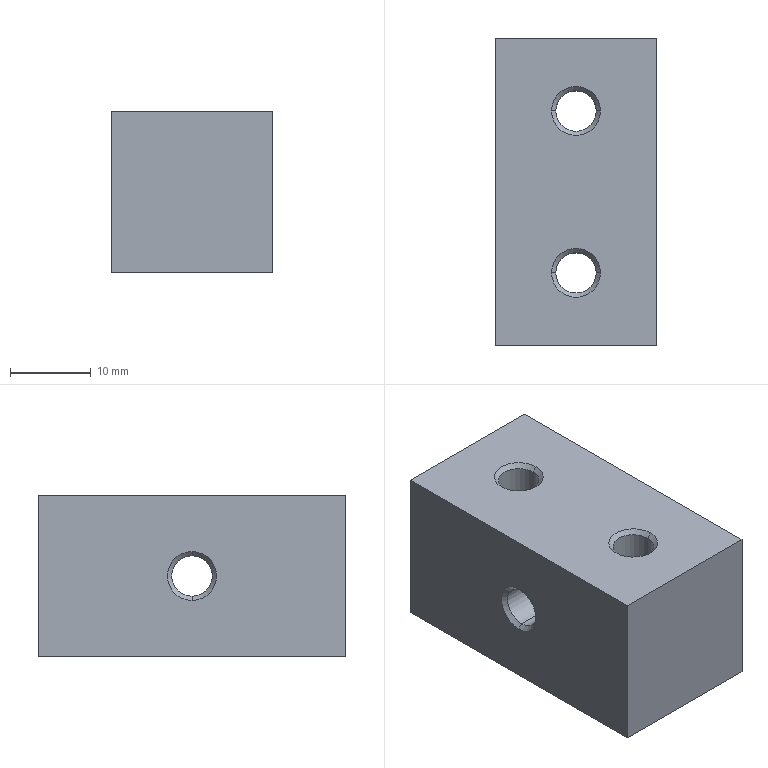Component | SolidWorks | NameDuplicate-1SupportBlock-2 | 1 solid | 18 faces | box 20 x 38 x 20 mm | volume 14015 mm3 | cone 6 | cylinder 6 | plane 6 | commonest cylinder face diameters 5 x6
build123d program:
from build123d import *

# Parameters (mm, degrees)
SKETCH1_W                = 20
SKETCH1_H                = 38
BOSS_EXTRUDE1_DEPTH      = 20
F_5_0_5_DIAMETER_HOLE1_D = 5
F_5_0_5_DIAMETER_HOLE2_D = 5
CHAMFER1_SIZE            = 0.525


with BuildPart() as part:
    # Sketch1 → Boss-Extrude1 (new body)
    with BuildSketch(Plane(origin=(10, 0, 0), x_dir=(0, 0, -1), z_dir=(1, 0, 0))):
        Rectangle(SKETCH1_W, SKETCH1_H)
    extrude(amount=-BOSS_EXTRUDE1_DEPTH)

    # 5.0 _5_ Diameter Hole1 (through all)
    with Locations(Plane(origin=(10, 0, 0), x_dir=(0, 0, -1), z_dir=(1, 0, 0))):
        with Locations((0, 0)):
            Hole(F_5_0_5_DIAMETER_HOLE1_D / 2)

    # 5.0 _5_ Diameter Hole2 (through all)
    with Locations(Plane.XY.offset(10)):
        with Locations((0, -10), (0, 10)):
            Hole(F_5_0_5_DIAMETER_HOLE2_D / 2)

    # Chamfer1
    chamfer1_edges = [part.edges().sort_by_distance(p)[0] for p in [
        (10, 0, -2.5),
        (2.5, 10, 10),
        (2.5, -10, 10),
    ]]
    chamfer(chamfer1_edges, length=CHAMFER1_SIZE)


solid = part.part

# Placed as in the assembly
solid = solid.moved(Location((-387, 406, -252.5), (0, 0, 180)))
STEP:
#1=COLOUR_RGB('',0.7922,0.8196,0.9333);
#2=FILL_AREA_STYLE_COLOUR('',#1);
#3=FILL_AREA_STYLE('',(#2));
#4=SURFACE_STYLE_FILL_AREA(#3);
#5=SURFACE_SIDE_STYLE('',(#4));
#6=SURFACE_STYLE_USAGE(.BOTH.,#5);
#7=PRESENTATION_STYLE_ASSIGNMENT((#6));
#8=CARTESIAN_POINT('',(-15.138,16.378,-9.568));
#9=VERTEX_POINT('',#8);
#10=CARTESIAN_POINT('',(-15.335,16.378,-9.568));
#11=VERTEX_POINT('',#10);
#12=CARTESIAN_POINT('',(-15.236,16.378,-9.568));
#13=DIRECTION('',(0.,0.,1.));
#14=DIRECTION('',(-1.,0.,0.));
#15=AXIS2_PLACEMENT_3D('',#12,#13,#14);
#16=CIRCLE('',#15,0.09843);
#17=EDGE_CURVE('',#9,#11,#16,.T.);
#18=ORIENTED_EDGE('',*,*,#17,.F.);
#19=CARTESIAN_POINT('',(-15.117,16.378,-9.547));
#20=VERTEX_POINT('',#19);
#21=CARTESIAN_POINT('',(-15.138,16.378,-9.568));
#22=DIRECTION('',(0.7071,0.,0.7071));
#23=VECTOR('',#22,39.37);
#24=LINE('',#21,#23);
#25=EDGE_CURVE('',#9,#20,#24,.T.);
#26=ORIENTED_EDGE('',*,*,#25,.T.);
#27=CARTESIAN_POINT('',(-15.355,16.378,-9.547));
#28=VERTEX_POINT('',#27);
#29=CARTESIAN_POINT('',(-15.236,16.378,-9.547));
#30=DIRECTION('',(-0.,-0.,-1.));
#31=DIRECTION('',(-1.,0.,0.));
#32=AXIS2_PLACEMENT_3D('',#29,#30,#31);
#33=CIRCLE('',#32,0.1191);
#34=EDGE_CURVE('',#28,#20,#33,.T.);
#35=ORIENTED_EDGE('',*,*,#34,.F.);
#36=CARTESIAN_POINT('',(-15.335,16.378,-9.568));
#37=DIRECTION('',(-0.7071,-0.,0.7071));
#38=VECTOR('',#37,39.37);
#39=LINE('',#36,#38);
#40=EDGE_CURVE('',#11,#28,#39,.T.);
#41=ORIENTED_EDGE('',*,*,#40,.F.);
#42=EDGE_LOOP('',(#18,#26,#35,#41));
#43=FACE_OUTER_BOUND('',#42,.T.);
#44=CARTESIAN_POINT('',(-15.236,16.378,-9.568));
#45=DIRECTION('',(0.,0.,1.));
#46=DIRECTION('',(-1.,0.,0.));
#47=AXIS2_PLACEMENT_3D('',#44,#45,#46);
#48=CONICAL_SURFACE('',#47,0.09843,0.7854);
#49=ADVANCED_FACE('',(#43),#48,.F.);
#50=CARTESIAN_POINT('',(-15.609,15.984,-9.843));
#51=VERTEX_POINT('',#50);
#52=CARTESIAN_POINT('',(-15.609,15.984,-10.039));
#53=VERTEX_POINT('',#52);
#54=CARTESIAN_POINT('',(-15.609,15.984,-9.941));
#55=DIRECTION('',(-1.,-0.,0.));
#56=DIRECTION('',(0.,0.,-1.));
#57=AXIS2_PLACEMENT_3D('',#54,#55,#56);
#58=CIRCLE('',#57,0.09843);
#59=EDGE_CURVE('',#51,#53,#58,.T.);
#60=ORIENTED_EDGE('',*,*,#59,.F.);
#61=CARTESIAN_POINT('',(-15.63,15.984,-9.822));
#62=VERTEX_POINT('',#61);
#63=CARTESIAN_POINT('',(-15.609,15.984,-9.843));
#64=DIRECTION('',(-0.7071,-0.,0.7071));
#65=VECTOR('',#64,39.37);
#66=LINE('',#63,#65);
#67=EDGE_CURVE('',#51,#62,#66,.T.);
#68=ORIENTED_EDGE('',*,*,#67,.T.);
#69=CARTESIAN_POINT('',(-15.63,15.984,-10.06));
#70=VERTEX_POINT('',#69);
#71=CARTESIAN_POINT('',(-15.63,15.984,-9.941));
#72=DIRECTION('',(1.,0.,-0.));
#73=DIRECTION('',(0.,0.,-1.));
#74=AXIS2_PLACEMENT_3D('',#71,#72,#73);
#75=CIRCLE('',#74,0.1191);
#76=EDGE_CURVE('',#70,#62,#75,.T.);
#77=ORIENTED_EDGE('',*,*,#76,.F.);
#78=CARTESIAN_POINT('',(-15.609,15.984,-10.039));
#79=DIRECTION('',(-0.7071,-0.,-0.7071));
#80=VECTOR('',#79,39.37);
#81=LINE('',#78,#80);
#82=EDGE_CURVE('',#53,#70,#81,.T.);
#83=ORIENTED_EDGE('',*,*,#82,.F.);
#84=EDGE_LOOP('',(#60,#68,#77,#83));
#85=FACE_OUTER_BOUND('',#84,.T.);
#86=CARTESIAN_POINT('',(-15.609,15.984,-9.941));
#87=DIRECTION('',(-1.,-0.,0.));
#88=DIRECTION('',(0.,0.,-1.));
#89=AXIS2_PLACEMENT_3D('',#86,#87,#88);
#90=CONICAL_SURFACE('',#89,0.09843,0.7854);
#91=ADVANCED_FACE('',(#85),#90,.F.);
#92=CARTESIAN_POINT('',(-15.138,15.591,-9.568));
#93=VERTEX_POINT('',#92);
#94=CARTESIAN_POINT('',(-15.335,15.591,-9.568));
#95=VERTEX_POINT('',#94);
#96=CARTESIAN_POINT('',(-15.236,15.591,-9.568));
#97=DIRECTION('',(0.,0.,1.));
#98=DIRECTION('',(-1.,0.,0.));
#99=AXIS2_PLACEMENT_3D('',#96,#97,#98);
#100=CIRCLE('',#99,0.09843);
#101=EDGE_CURVE('',#93,#95,#100,.T.);
#102=ORIENTED_EDGE('',*,*,#101,.F.);
#103=CARTESIAN_POINT('',(-15.117,15.591,-9.547));
#104=VERTEX_POINT('',#103);
#105=CARTESIAN_POINT('',(-15.138,15.591,-9.568));
#106=DIRECTION('',(0.7071,0.,0.7071));
#107=VECTOR('',#106,39.37);
#108=LINE('',#105,#107);
#109=EDGE_CURVE('',#93,#104,#108,.T.);
#110=ORIENTED_EDGE('',*,*,#109,.T.);
#111=CARTESIAN_POINT('',(-15.355,15.591,-9.547));
#112=VERTEX_POINT('',#111);
#113=CARTESIAN_POINT('',(-15.236,15.591,-9.547));
#114=DIRECTION('',(-0.,-0.,-1.));
#115=DIRECTION('',(-1.,0.,0.));
#116=AXIS2_PLACEMENT_3D('',#113,#114,#115);
#117=CIRCLE('',#116,0.1191);
#118=EDGE_CURVE('',#112,#104,#117,.T.);
#119=ORIENTED_EDGE('',*,*,#118,.F.);
#120=CARTESIAN_POINT('',(-15.335,15.591,-9.568));
#121=DIRECTION('',(-0.7071,-0.,0.7071));
#122=VECTOR('',#121,39.37);
#123=LINE('',#120,#122);
#124=EDGE_CURVE('',#95,#112,#123,.T.);
#125=ORIENTED_EDGE('',*,*,#124,.F.);
#126=EDGE_LOOP('',(#102,#110,#119,#125));
#127=FACE_OUTER_BOUND('',#126,.T.);
#128=CARTESIAN_POINT('',(-15.236,15.591,-9.568));
#129=DIRECTION('',(0.,0.,1.));
#130=DIRECTION('',(-1.,0.,0.));
#131=AXIS2_PLACEMENT_3D('',#128,#129,#130);
#132=CONICAL_SURFACE('',#131,0.09843,0.7854);
#133=ADVANCED_FACE('',(#127),#132,.F.);
#134=CARTESIAN_POINT('',(-15.138,16.378,-10.335));
#135=VERTEX_POINT('',#134);
#136=CARTESIAN_POINT('',(-15.335,16.378,-10.335));
#137=VERTEX_POINT('',#136);
#138=CARTESIAN_POINT('',(-15.236,16.378,-10.335));
#139=DIRECTION('',(0.,0.,1.));
#140=DIRECTION('',(-1.,0.,0.));
#141=AXIS2_PLACEMENT_3D('',#138,#139,#140);
#142=CIRCLE('',#141,0.09843);
#143=EDGE_CURVE('',#135,#137,#142,.T.);
#144=ORIENTED_EDGE('',*,*,#143,.F.);
#145=CARTESIAN_POINT('',(-15.138,16.378,-9.547));
#146=DIRECTION('',(0.,0.,1.));
#147=VECTOR('',#146,39.37);
#148=LINE('',#145,#147);
#149=EDGE_CURVE('',#135,#9,#148,.T.);
#150=ORIENTED_EDGE('',*,*,#149,.T.);
#151=ORIENTED_EDGE('',*,*,#17,.T.);
#152=CARTESIAN_POINT('',(-15.335,16.378,-9.547));
#153=DIRECTION('',(0.,0.,1.));
#154=VECTOR('',#153,39.37);
#155=LINE('',#152,#154);
#156=EDGE_CURVE('',#137,#11,#155,.T.);
#157=ORIENTED_EDGE('',*,*,#156,.F.);
#158=EDGE_LOOP('',(#144,#150,#151,#157));
#159=FACE_OUTER_BOUND('',#158,.T.);
#160=CARTESIAN_POINT('',(-15.236,16.378,-9.547));
#161=DIRECTION('',(0.,0.,1.));
#162=DIRECTION('',(-1.,0.,0.));
#163=AXIS2_PLACEMENT_3D('',#160,#161,#162);
#164=CYLINDRICAL_SURFACE('',#163,0.09843);
#165=ADVANCED_FACE('',(#159),#164,.F.);
#166=CARTESIAN_POINT('',(-15.138,15.591,-10.335));
#167=VERTEX_POINT('',#166);
#168=CARTESIAN_POINT('',(-15.335,15.591,-10.335));
#169=VERTEX_POINT('',#168);
#170=CARTESIAN_POINT('',(-15.236,15.591,-10.335));
#171=DIRECTION('',(0.,0.,1.));
#172=DIRECTION('',(-1.,0.,0.));
#173=AXIS2_PLACEMENT_3D('',#170,#171,#172);
#174=CIRCLE('',#173,0.09843);
#175=EDGE_CURVE('',#167,#169,#174,.T.);
#176=ORIENTED_EDGE('',*,*,#175,.F.);
#177=CARTESIAN_POINT('',(-15.138,15.591,-9.547));
#178=DIRECTION('',(0.,0.,1.));
#179=VECTOR('',#178,39.37);
#180=LINE('',#177,#179);
#181=EDGE_CURVE('',#167,#93,#180,.T.);
#182=ORIENTED_EDGE('',*,*,#181,.T.);
#183=ORIENTED_EDGE('',*,*,#101,.T.);
#184=CARTESIAN_POINT('',(-15.335,15.591,-9.547));
#185=DIRECTION('',(0.,0.,1.));
#186=VECTOR('',#185,39.37);
#187=LINE('',#184,#186);
#188=EDGE_CURVE('',#169,#95,#187,.T.);
#189=ORIENTED_EDGE('',*,*,#188,.F.);
#190=EDGE_LOOP('',(#176,#182,#183,#189));
#191=FACE_OUTER_BOUND('',#190,.T.);
#192=CARTESIAN_POINT('',(-15.236,15.591,-9.547));
#193=DIRECTION('',(0.,0.,1.));
#194=DIRECTION('',(-1.,0.,0.));
#195=AXIS2_PLACEMENT_3D('',#192,#193,#194);
#196=CYLINDRICAL_SURFACE('',#195,0.09843);
#197=ADVANCED_FACE('',(#191),#196,.F.);
#198=CARTESIAN_POINT('',(-14.843,15.984,-9.843));
#199=VERTEX_POINT('',#198);
#200=CARTESIAN_POINT('',(-14.843,15.984,-10.039));
#201=VERTEX_POINT('',#200);
#202=CARTESIAN_POINT('',(-14.843,15.984,-9.941));
#203=DIRECTION('',(-1.,-0.,0.));
#204=DIRECTION('',(0.,0.,-1.));
#205=AXIS2_PLACEMENT_3D('',#202,#203,#204);
#206=CIRCLE('',#205,0.09843);
#207=EDGE_CURVE('',#199,#201,#206,.T.);
#208=ORIENTED_EDGE('',*,*,#207,.F.);
#209=CARTESIAN_POINT('',(-15.63,15.984,-9.843));
#210=DIRECTION('',(-1.,-0.,0.));
#211=VECTOR('',#210,39.37);
#212=LINE('',#209,#211);
#213=EDGE_CURVE('',#199,#51,#212,.T.);
#214=ORIENTED_EDGE('',*,*,#213,.T.);
#215=ORIENTED_EDGE('',*,*,#59,.T.);
#216=CARTESIAN_POINT('',(-15.63,15.984,-10.039));
#217=DIRECTION('',(-1.,-0.,0.));
#218=VECTOR('',#217,39.37);
#219=LINE('',#216,#218);
#220=EDGE_CURVE('',#201,#53,#219,.T.);
#221=ORIENTED_EDGE('',*,*,#220,.F.);
#222=EDGE_LOOP('',(#208,#214,#215,#221));
#223=FACE_OUTER_BOUND('',#222,.T.);
#224=CARTESIAN_POINT('',(-15.63,15.984,-9.941));
#225=DIRECTION('',(-1.,-0.,0.));
#226=DIRECTION('',(0.,0.,-1.));
#227=AXIS2_PLACEMENT_3D('',#224,#225,#226);
#228=CYLINDRICAL_SURFACE('',#227,0.09843);
#229=ADVANCED_FACE('',(#223),#228,.F.);
#230=CARTESIAN_POINT('',(-15.63,15.236,-10.335));
#231=VERTEX_POINT('',#230);
#232=CARTESIAN_POINT('',(-15.63,15.236,-9.547));
#233=VERTEX_POINT('',#232);
#234=CARTESIAN_POINT('',(-15.63,15.236,-10.335));
#235=DIRECTION('',(0.,0.,1.));
#236=VECTOR('',#235,39.37);
#237=LINE('',#234,#236);
#238=EDGE_CURVE('',#231,#233,#237,.T.);
#239=ORIENTED_EDGE('',*,*,#238,.F.);
#240=CARTESIAN_POINT('',(-14.843,15.236,-10.335));
#241=VERTEX_POINT('',#240);
#242=CARTESIAN_POINT('',(-14.843,15.236,-10.335));
#243=DIRECTION('',(-1.,-0.,0.));
#244=VECTOR('',#243,39.37);
#245=LINE('',#242,#244);
#246=EDGE_CURVE('',#241,#231,#245,.T.);
#247=ORIENTED_EDGE('',*,*,#246,.F.);
#248=CARTESIAN_POINT('',(-14.843,15.236,-9.547));
#249=VERTEX_POINT('',#248);
#250=CARTESIAN_POINT('',(-14.843,15.236,-10.335));
#251=DIRECTION('',(0.,0.,1.));
#252=VECTOR('',#251,39.37);
#253=LINE('',#250,#252);
#254=EDGE_CURVE('',#241,#249,#253,.T.);
#255=ORIENTED_EDGE('',*,*,#254,.T.);
#256=CARTESIAN_POINT('',(-14.843,15.236,-9.547));
#257=DIRECTION('',(-1.,-0.,0.));
#258=VECTOR('',#257,39.37);
#259=LINE('',#256,#258);
#260=EDGE_CURVE('',#249,#233,#259,.T.);
#261=ORIENTED_EDGE('',*,*,#260,.T.);
#262=EDGE_LOOP('',(#239,#247,#255,#261));
#263=FACE_OUTER_BOUND('',#262,.T.);
#264=CARTESIAN_POINT('',(-14.843,15.236,-10.335));
#265=DIRECTION('',(0.,-1.,0.));
#266=DIRECTION('',(0.,0.,1.));
#267=AXIS2_PLACEMENT_3D('',#264,#265,#266);
#268=PLANE('',#267);
#269=ADVANCED_FACE('',(#263),#268,.T.);
#270=CARTESIAN_POINT('',(-15.236,16.378,-10.335));
#271=DIRECTION('',(0.,0.,1.));
#272=DIRECTION('',(-1.,0.,0.));
#273=AXIS2_PLACEMENT_3D('',#270,#271,#272);
#274=CIRCLE('',#273,0.09843);
#275=EDGE_CURVE('',#137,#135,#274,.T.);
#276=ORIENTED_EDGE('',*,*,#275,.T.);
#277=ORIENTED_EDGE('',*,*,#143,.T.);
#278=EDGE_LOOP('',(#276,#277));
#279=FACE_BOUND('',#278,.T.);
#280=CARTESIAN_POINT('',(-15.236,15.591,-10.335));
#281=DIRECTION('',(0.,0.,1.));
#282=DIRECTION('',(-1.,0.,0.));
#283=AXIS2_PLACEMENT_3D('',#280,#281,#282);
#284=CIRCLE('',#283,0.09843);
#285=EDGE_CURVE('',#169,#167,#284,.T.);
#286=ORIENTED_EDGE('',*,*,#285,.T.);
#287=ORIENTED_EDGE('',*,*,#175,.T.);
#288=EDGE_LOOP('',(#286,#287));
#289=FACE_BOUND('',#288,.T.);
#290=CARTESIAN_POINT('',(-15.63,16.732,-10.335));
#291=VERTEX_POINT('',#290);
#292=CARTESIAN_POINT('',(-15.63,16.732,-10.335));
#293=DIRECTION('',(0.,-1.,0.));
#294=VECTOR('',#293,39.37);
#295=LINE('',#292,#294);
#296=EDGE_CURVE('',#291,#231,#295,.T.);
#297=ORIENTED_EDGE('',*,*,#296,.F.);
#298=CARTESIAN_POINT('',(-14.843,16.732,-10.335));
#299=VERTEX_POINT('',#298);
#300=CARTESIAN_POINT('',(-14.843,16.732,-10.335));
#301=DIRECTION('',(-1.,-0.,0.));
#302=VECTOR('',#301,39.37);
#303=LINE('',#300,#302);
#304=EDGE_CURVE('',#299,#291,#303,.T.);
#305=ORIENTED_EDGE('',*,*,#304,.F.);
#306=CARTESIAN_POINT('',(-14.843,16.732,-10.335));
#307=DIRECTION('',(0.,-1.,0.));
#308=VECTOR('',#307,39.37);
#309=LINE('',#306,#308);
#310=EDGE_CURVE('',#299,#241,#309,.T.);
#311=ORIENTED_EDGE('',*,*,#310,.T.);
#312=ORIENTED_EDGE('',*,*,#246,.T.);
#313=EDGE_LOOP('',(#297,#305,#311,#312));
#314=FACE_OUTER_BOUND('',#313,.T.);
#315=CARTESIAN_POINT('',(-14.843,16.732,-10.335));
#316=DIRECTION('',(-0.,-0.,-1.));
#317=DIRECTION('',(1.,0.,-0.));
#318=AXIS2_PLACEMENT_3D('',#315,#316,#317);
#319=PLANE('',#318);
#320=ADVANCED_FACE('',(#279,#289,#314),#319,.T.);
#321=CARTESIAN_POINT('',(-15.63,16.732,-9.547));
#322=VERTEX_POINT('',#321);
#323=CARTESIAN_POINT('',(-15.63,16.732,-9.547));
#324=DIRECTION('',(-0.,-0.,-1.));
#325=VECTOR('',#324,39.37);
#326=LINE('',#323,#325);
#327=EDGE_CURVE('',#322,#291,#326,.T.);
#328=ORIENTED_EDGE('',*,*,#327,.F.);
#329=CARTESIAN_POINT('',(-14.843,16.732,-9.547));
#330=VERTEX_POINT('',#329);
#331=CARTESIAN_POINT('',(-14.843,16.732,-9.547));
#332=DIRECTION('',(-1.,-0.,0.));
#333=VECTOR('',#332,39.37);
#334=LINE('',#331,#333);
#335=EDGE_CURVE('',#330,#322,#334,.T.);
#336=ORIENTED_EDGE('',*,*,#335,.F.);
#337=CARTESIAN_POINT('',(-14.843,16.732,-9.547));
#338=DIRECTION('',(-0.,-0.,-1.));
#339=VECTOR('',#338,39.37);
#340=LINE('',#337,#339);
#341=EDGE_CURVE('',#330,#299,#340,.T.);
#342=ORIENTED_EDGE('',*,*,#341,.T.);
#343=ORIENTED_EDGE('',*,*,#304,.T.);
#344=EDGE_LOOP('',(#328,#336,#342,#343));
#345=FACE_OUTER_BOUND('',#344,.T.);
#346=CARTESIAN_POINT('',(-14.843,16.732,-9.547));
#347=DIRECTION('',(-0.,1.,-0.));
#348=DIRECTION('',(-0.,-0.,-1.));
#349=AXIS2_PLACEMENT_3D('',#346,#347,#348);
#350=PLANE('',#349);
#351=ADVANCED_FACE('',(#345),#350,.T.);
#352=ORIENTED_EDGE('',*,*,#118,.T.);
#353=CARTESIAN_POINT('',(-15.236,15.591,-9.547));
#354=DIRECTION('',(-0.,-0.,-1.));
#355=DIRECTION('',(-1.,0.,0.));
#356=AXIS2_PLACEMENT_3D('',#353,#354,#355);
#357=CIRCLE('',#356,0.1191);
#358=EDGE_CURVE('',#104,#112,#357,.T.);
#359=ORIENTED_EDGE('',*,*,#358,.T.);
#360=EDGE_LOOP('',(#352,#359));
#361=FACE_BOUND('',#360,.T.);
#362=ORIENTED_EDGE('',*,*,#34,.T.);
#363=CARTESIAN_POINT('',(-15.236,16.378,-9.547));
#364=DIRECTION('',(-0.,-0.,-1.));
#365=DIRECTION('',(-1.,0.,0.));
#366=AXIS2_PLACEMENT_3D('',#363,#364,#365);
#367=CIRCLE('',#366,0.1191);
#368=EDGE_CURVE('',#20,#28,#367,.T.);
#369=ORIENTED_EDGE('',*,*,#368,.T.);
#370=EDGE_LOOP('',(#362,#369));
#371=FACE_BOUND('',#370,.T.);
#372=CARTESIAN_POINT('',(-15.63,15.236,-9.547));
#373=DIRECTION('',(-0.,1.,-0.));
#374=VECTOR('',#373,39.37);
#375=LINE('',#372,#374);
#376=EDGE_CURVE('',#233,#322,#375,.T.);
#377=ORIENTED_EDGE('',*,*,#376,.F.);
#378=ORIENTED_EDGE('',*,*,#260,.F.);
#379=CARTESIAN_POINT('',(-14.843,15.236,-9.547));
#380=DIRECTION('',(-0.,1.,-0.));
#381=VECTOR('',#380,39.37);
#382=LINE('',#379,#381);
#383=EDGE_CURVE('',#249,#330,#382,.T.);
#384=ORIENTED_EDGE('',*,*,#383,.T.);
#385=ORIENTED_EDGE('',*,*,#335,.T.);
#386=EDGE_LOOP('',(#377,#378,#384,#385));
#387=FACE_OUTER_BOUND('',#386,.T.);
#388=CARTESIAN_POINT('',(-14.843,15.236,-9.547));
#389=DIRECTION('',(0.,0.,1.));
#390=DIRECTION('',(-1.,-0.,0.));
#391=AXIS2_PLACEMENT_3D('',#388,#389,#390);
#392=PLANE('',#391);
#393=ADVANCED_FACE('',(#361,#371,#387),#392,.T.);
#394=CARTESIAN_POINT('',(-14.843,15.984,-9.941));
#395=DIRECTION('',(-1.,-0.,0.));
#396=DIRECTION('',(0.,0.,-1.));
#397=AXIS2_PLACEMENT_3D('',#394,#395,#396);
#398=CIRCLE('',#397,0.09843);
#399=EDGE_CURVE('',#201,#199,#398,.T.);
#400=ORIENTED_EDGE('',*,*,#399,.T.);
#401=ORIENTED_EDGE('',*,*,#207,.T.);
#402=EDGE_LOOP('',(#400,#401));
#403=FACE_BOUND('',#402,.T.);
#404=ORIENTED_EDGE('',*,*,#254,.F.);
#405=ORIENTED_EDGE('',*,*,#310,.F.);
#406=ORIENTED_EDGE('',*,*,#341,.F.);
#407=ORIENTED_EDGE('',*,*,#383,.F.);
#408=EDGE_LOOP('',(#404,#405,#406,#407));
#409=FACE_OUTER_BOUND('',#408,.T.);
#410=CARTESIAN_POINT('',(-14.843,15.984,-9.941));
#411=DIRECTION('',(-1.,-0.,0.));
#412=DIRECTION('',(-0.,-0.,-1.));
#413=AXIS2_PLACEMENT_3D('',#410,#411,#412);
#414=PLANE('',#413);
#415=ADVANCED_FACE('',(#403,#409),#414,.F.);
#416=ORIENTED_EDGE('',*,*,#76,.T.);
#417=CARTESIAN_POINT('',(-15.63,15.984,-9.941));
#418=DIRECTION('',(1.,0.,-0.));
#419=DIRECTION('',(0.,0.,-1.));
#420=AXIS2_PLACEMENT_3D('',#417,#418,#419);
#421=CIRCLE('',#420,0.1191);
#422=EDGE_CURVE('',#62,#70,#421,.T.);
#423=ORIENTED_EDGE('',*,*,#422,.T.);
#424=EDGE_LOOP('',(#416,#423));
#425=FACE_BOUND('',#424,.T.);
#426=ORIENTED_EDGE('',*,*,#238,.T.);
#427=ORIENTED_EDGE('',*,*,#376,.T.);
#428=ORIENTED_EDGE('',*,*,#327,.T.);
#429=ORIENTED_EDGE('',*,*,#296,.T.);
#430=EDGE_LOOP('',(#426,#427,#428,#429));
#431=FACE_OUTER_BOUND('',#430,.T.);
#432=CARTESIAN_POINT('',(-15.63,15.984,-9.941));
#433=DIRECTION('',(-1.,-0.,0.));
#434=DIRECTION('',(-0.,-0.,-1.));
#435=AXIS2_PLACEMENT_3D('',#432,#433,#434);
#436=PLANE('',#435);
#437=ADVANCED_FACE('',(#425,#431),#436,.T.);
#438=ORIENTED_EDGE('',*,*,#213,.F.);
#439=ORIENTED_EDGE('',*,*,#399,.F.);
#440=ORIENTED_EDGE('',*,*,#220,.T.);
#441=CARTESIAN_POINT('',(-15.609,15.984,-9.941));
#442=DIRECTION('',(-1.,-0.,0.));
#443=DIRECTION('',(0.,0.,-1.));
#444=AXIS2_PLACEMENT_3D('',#441,#442,#443);
#445=CIRCLE('',#444,0.09843);
#446=EDGE_CURVE('',#53,#51,#445,.T.);
#447=ORIENTED_EDGE('',*,*,#446,.T.);
#448=EDGE_LOOP('',(#438,#439,#440,#447));
#449=FACE_OUTER_BOUND('',#448,.T.);
#450=CARTESIAN_POINT('',(-15.63,15.984,-9.941));
#451=DIRECTION('',(-1.,-0.,0.));
#452=DIRECTION('',(0.,0.,-1.));
#453=AXIS2_PLACEMENT_3D('',#450,#451,#452);
#454=CYLINDRICAL_SURFACE('',#453,0.09843);
#455=ADVANCED_FACE('',(#449),#454,.F.);
#456=ORIENTED_EDGE('',*,*,#181,.F.);
#457=ORIENTED_EDGE('',*,*,#285,.F.);
#458=ORIENTED_EDGE('',*,*,#188,.T.);
#459=CARTESIAN_POINT('',(-15.236,15.591,-9.568));
#460=DIRECTION('',(0.,0.,1.));
#461=DIRECTION('',(-1.,0.,0.));
#462=AXIS2_PLACEMENT_3D('',#459,#460,#461);
#463=CIRCLE('',#462,0.09843);
#464=EDGE_CURVE('',#95,#93,#463,.T.);
#465=ORIENTED_EDGE('',*,*,#464,.T.);
#466=EDGE_LOOP('',(#456,#457,#458,#465));
#467=FACE_OUTER_BOUND('',#466,.T.);
#468=CARTESIAN_POINT('',(-15.236,15.591,-9.547));
#469=DIRECTION('',(0.,0.,1.));
#470=DIRECTION('',(-1.,0.,0.));
#471=AXIS2_PLACEMENT_3D('',#468,#469,#470);
#472=CYLINDRICAL_SURFACE('',#471,0.09843);
#473=ADVANCED_FACE('',(#467),#472,.F.);
#474=ORIENTED_EDGE('',*,*,#149,.F.);
#475=ORIENTED_EDGE('',*,*,#275,.F.);
#476=ORIENTED_EDGE('',*,*,#156,.T.);
#477=CARTESIAN_POINT('',(-15.236,16.378,-9.568));
#478=DIRECTION('',(0.,0.,1.));
#479=DIRECTION('',(-1.,0.,0.));
#480=AXIS2_PLACEMENT_3D('',#477,#478,#479);
#481=CIRCLE('',#480,0.09843);
#482=EDGE_CURVE('',#11,#9,#481,.T.);
#483=ORIENTED_EDGE('',*,*,#482,.T.);
#484=EDGE_LOOP('',(#474,#475,#476,#483));
#485=FACE_OUTER_BOUND('',#484,.T.);
#486=CARTESIAN_POINT('',(-15.236,16.378,-9.547));
#487=DIRECTION('',(0.,0.,1.));
#488=DIRECTION('',(-1.,0.,0.));
#489=AXIS2_PLACEMENT_3D('',#486,#487,#488);
#490=CYLINDRICAL_SURFACE('',#489,0.09843);
#491=ADVANCED_FACE('',(#485),#490,.F.);
#492=ORIENTED_EDGE('',*,*,#109,.F.);
#493=ORIENTED_EDGE('',*,*,#464,.F.);
#494=ORIENTED_EDGE('',*,*,#124,.T.);
#495=ORIENTED_EDGE('',*,*,#358,.F.);
#496=EDGE_LOOP('',(#492,#493,#494,#495));
#497=FACE_OUTER_BOUND('',#496,.T.);
#498=CARTESIAN_POINT('',(-15.236,15.591,-9.568));
#499=DIRECTION('',(0.,0.,1.));
#500=DIRECTION('',(-1.,0.,0.));
#501=AXIS2_PLACEMENT_3D('',#498,#499,#500);
#502=CONICAL_SURFACE('',#501,0.09843,0.7854);
#503=ADVANCED_FACE('',(#497),#502,.F.);
#504=ORIENTED_EDGE('',*,*,#67,.F.);
#505=ORIENTED_EDGE('',*,*,#446,.F.);
#506=ORIENTED_EDGE('',*,*,#82,.T.);
#507=ORIENTED_EDGE('',*,*,#422,.F.);
#508=EDGE_LOOP('',(#504,#505,#506,#507));
#509=FACE_OUTER_BOUND('',#508,.T.);
#510=CARTESIAN_POINT('',(-15.609,15.984,-9.941));
#511=DIRECTION('',(-1.,-0.,0.));
#512=DIRECTION('',(0.,0.,-1.));
#513=AXIS2_PLACEMENT_3D('',#510,#511,#512);
#514=CONICAL_SURFACE('',#513,0.09843,0.7854);
#515=ADVANCED_FACE('',(#509),#514,.F.);
#516=ORIENTED_EDGE('',*,*,#25,.F.);
#517=ORIENTED_EDGE('',*,*,#482,.F.);
#518=ORIENTED_EDGE('',*,*,#40,.T.);
#519=ORIENTED_EDGE('',*,*,#368,.F.);
#520=EDGE_LOOP('',(#516,#517,#518,#519));
#521=FACE_OUTER_BOUND('',#520,.T.);
#522=CARTESIAN_POINT('',(-15.236,16.378,-9.568));
#523=DIRECTION('',(0.,0.,1.));
#524=DIRECTION('',(-1.,0.,0.));
#525=AXIS2_PLACEMENT_3D('',#522,#523,#524);
#526=CONICAL_SURFACE('',#525,0.09843,0.7854);
#527=ADVANCED_FACE('',(#521),#526,.F.);
#528=CLOSED_SHELL('',(#49,#91,#133,#165,#197,#229,#269,#320,#351,#393,#415,#437,#455,#473,#491,#503,#515,#527));
#529=MANIFOLD_SOLID_BREP('',#528);
#530=STYLED_ITEM('',(#7),#529);
#531=PRESENTATION_LAYER_ASSIGNMENT('','',(#530));
#532=(LENGTH_UNIT()NAMED_UNIT(*)SI_UNIT($,.METRE.));
#533=LENGTH_MEASURE_WITH_UNIT(LENGTH_MEASURE(0.0254),#532);
#534=DIMENSIONAL_EXPONENTS(1.,0.,0.,0.,0.,0.,0.);
#535=(CONVERSION_BASED_UNIT('',#533)LENGTH_UNIT()NAMED_UNIT(#534));
#536=UNCERTAINTY_MEASURE_WITH_UNIT(LENGTH_MEASURE(0.00001),#535,'','');
#537=(NAMED_UNIT(*)PLANE_ANGLE_UNIT()SI_UNIT($,.RADIAN.));
#538=(NAMED_UNIT(*)SI_UNIT($,.STERADIAN.)SOLID_ANGLE_UNIT());
#539=(GEOMETRIC_REPRESENTATION_CONTEXT(3)GLOBAL_UNCERTAINTY_ASSIGNED_CONTEXT((#536))GLOBAL_UNIT_ASSIGNED_CONTEXT((#535,#537,#538))REPRESENTATION_CONTEXT('',''));
#540=MECHANICAL_DESIGN_GEOMETRIC_PRESENTATION_REPRESENTATION('',(#530),#539);
#541=CARTESIAN_POINT('',(0.,0.,0.));
#542=DIRECTION('',(0.,0.,1.));
#543=DIRECTION('',(1.,0.,0.));
#544=AXIS2_PLACEMENT_3D('',#541,#542,#543);
#545=(LENGTH_UNIT()NAMED_UNIT(*)SI_UNIT($,.METRE.));
#546=LENGTH_MEASURE_WITH_UNIT(LENGTH_MEASURE(0.0254),#545);
#547=DIMENSIONAL_EXPONENTS(1.,0.,0.,0.,0.,0.,0.);
#548=(CONVERSION_BASED_UNIT('',#546)LENGTH_UNIT()NAMED_UNIT(#547));
#549=UNCERTAINTY_MEASURE_WITH_UNIT(LENGTH_MEASURE(0.00001),#548,'','');
#550=(NAMED_UNIT(*)PLANE_ANGLE_UNIT()SI_UNIT($,.RADIAN.));
#551=(NAMED_UNIT(*)SI_UNIT($,.STERADIAN.)SOLID_ANGLE_UNIT());
#552=(GEOMETRIC_REPRESENTATION_CONTEXT(3)GLOBAL_UNCERTAINTY_ASSIGNED_CONTEXT((#549))GLOBAL_UNIT_ASSIGNED_CONTEXT((#548,#550,#551))REPRESENTATION_CONTEXT('',''));
#553=ADVANCED_BREP_SHAPE_REPRESENTATION('',(#529,#544),#552);